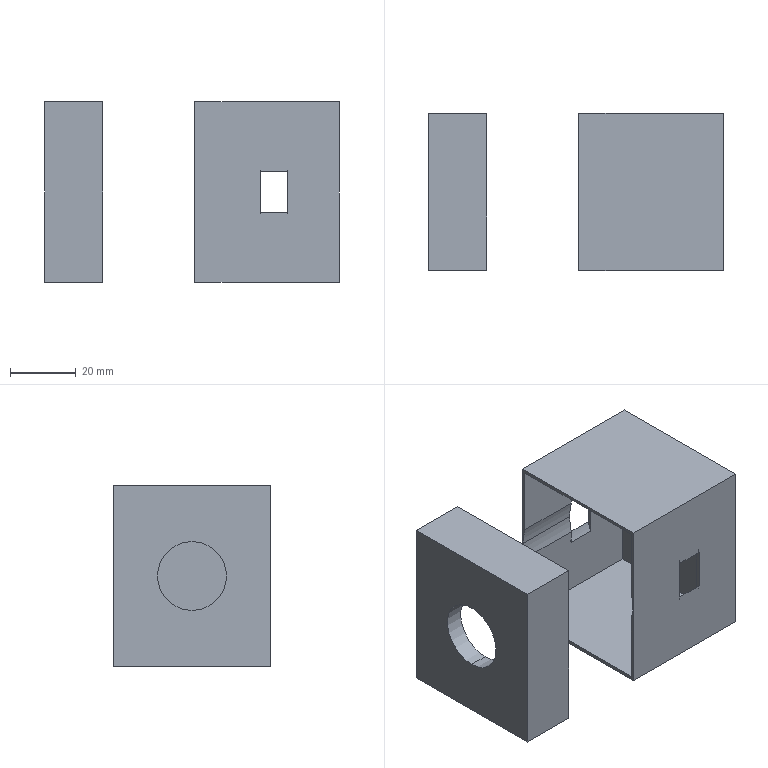Component | SolidWorks | BearingHousing-1 | 2 solids | 35 faces | box 89.77 x 47.79 x 55 mm | volume 28863 mm3 | plane 26 | cylinder 9 | commonest cylinder face diameters 49.4 x4 47.02 x3 21 x2
STEP:
#1=COLOUR_RGB('',0.7922,0.8196,0.9333);
#2=FILL_AREA_STYLE_COLOUR('',#1);
#3=FILL_AREA_STYLE('',(#2));
#4=SURFACE_STYLE_FILL_AREA(#3);
#5=SURFACE_SIDE_STYLE('',(#4));
#6=SURFACE_STYLE_USAGE(.BOTH.,#5);
#7=PRESENTATION_STYLE_ASSIGNMENT((#6));
#8=CARTESIAN_POINT('',(7.824,3.296,-0.0000003));
#9=VERTEX_POINT('',#8);
#10=CARTESIAN_POINT('',(7.824,3.272,-0.2103));
#11=VERTEX_POINT('',#10);
#12=CARTESIAN_POINT('',(7.824,2.371,-0.0000003));
#13=DIRECTION('',(-1.,-0.,-0.));
#14=DIRECTION('',(0.,-1.,-0.));
#15=AXIS2_PLACEMENT_3D('',#12,#13,#14);
#16=CIRCLE('',#15,0.9256);
#17=EDGE_CURVE('',#9,#11,#16,.T.);
#18=ORIENTED_EDGE('',*,*,#17,.F.);
#19=CARTESIAN_POINT('',(7.039,3.296,-0.0000003));
#20=VERTEX_POINT('',#19);
#21=CARTESIAN_POINT('',(7.826,3.296,-0.0000003));
#22=DIRECTION('',(-1.,-0.,-0.));
#23=VECTOR('',#22,39.37);
#24=LINE('',#21,#23);
#25=EDGE_CURVE('',#9,#20,#24,.T.);
#26=ORIENTED_EDGE('',*,*,#25,.T.);
#27=CARTESIAN_POINT('',(7.039,3.272,-0.2103));
#28=VERTEX_POINT('',#27);
#29=CARTESIAN_POINT('',(7.039,2.371,-0.0000003));
#30=DIRECTION('',(-1.,-0.,-0.));
#31=DIRECTION('',(0.,-1.,-0.));
#32=AXIS2_PLACEMENT_3D('',#29,#30,#31);
#33=CIRCLE('',#32,0.9256);
#34=EDGE_CURVE('',#20,#28,#33,.T.);
#35=ORIENTED_EDGE('',*,*,#34,.T.);
#36=CARTESIAN_POINT('',(7.826,3.272,-0.2103));
#37=DIRECTION('',(1.,0.,0.));
#38=VECTOR('',#37,39.37);
#39=LINE('',#36,#38);
#40=EDGE_CURVE('',#28,#11,#39,.T.);
#41=ORIENTED_EDGE('',*,*,#40,.T.);
#42=EDGE_LOOP('',(#18,#26,#35,#41));
#43=FACE_OUTER_BOUND('',#42,.T.);
#44=CARTESIAN_POINT('',(7.826,2.371,-0.0000003));
#45=DIRECTION('',(-1.,-0.,-0.));
#46=DIRECTION('',(0.,1.,0.));
#47=AXIS2_PLACEMENT_3D('',#44,#45,#46);
#48=CYLINDRICAL_SURFACE('',#47,0.9256);
#49=ADVANCED_FACE('',(#43),#48,.F.);
#50=CARTESIAN_POINT('',(7.039,1.469,0.2103));
#51=VERTEX_POINT('',#50);
#52=CARTESIAN_POINT('',(7.824,1.469,0.2103));
#53=VERTEX_POINT('',#52);
#54=CARTESIAN_POINT('',(7.826,1.469,0.2103));
#55=DIRECTION('',(1.,0.,0.));
#56=VECTOR('',#55,39.37);
#57=LINE('',#54,#56);
#58=EDGE_CURVE('',#51,#53,#57,.T.);
#59=ORIENTED_EDGE('',*,*,#58,.F.);
#60=CARTESIAN_POINT('',(7.039,1.469,1.043));
#61=VERTEX_POINT('',#60);
#62=CARTESIAN_POINT('',(7.039,1.469,0.8331));
#63=DIRECTION('',(0.,0.,-1.));
#64=VECTOR('',#63,39.37);
#65=LINE('',#62,#64);
#66=EDGE_CURVE('',#61,#51,#65,.T.);
#67=ORIENTED_EDGE('',*,*,#66,.F.);
#68=CARTESIAN_POINT('',(8.692,1.469,1.043));
#69=VERTEX_POINT('',#68);
#70=CARTESIAN_POINT('',(5.464,1.469,1.043));
#71=DIRECTION('',(1.,0.,0.));
#72=VECTOR('',#71,39.37);
#73=LINE('',#70,#72);
#74=EDGE_CURVE('',#61,#69,#73,.T.);
#75=ORIENTED_EDGE('',*,*,#74,.T.);
#76=CARTESIAN_POINT('',(8.692,1.469,-1.043));
#77=VERTEX_POINT('',#76);
#78=CARTESIAN_POINT('',(8.692,1.469,1.043));
#79=DIRECTION('',(0.,0.,-1.));
#80=VECTOR('',#79,39.37);
#81=LINE('',#78,#80);
#82=EDGE_CURVE('',#69,#77,#81,.T.);
#83=ORIENTED_EDGE('',*,*,#82,.T.);
#84=CARTESIAN_POINT('',(7.039,1.469,-1.043));
#85=VERTEX_POINT('',#84);
#86=CARTESIAN_POINT('',(5.464,1.469,-1.043));
#87=DIRECTION('',(1.,0.,0.));
#88=VECTOR('',#87,39.37);
#89=LINE('',#86,#88);
#90=EDGE_CURVE('',#85,#77,#89,.T.);
#91=ORIENTED_EDGE('',*,*,#90,.F.);
#92=CARTESIAN_POINT('',(7.039,1.469,-0.2103));
#93=VERTEX_POINT('',#92);
#94=CARTESIAN_POINT('',(7.039,1.469,0.8331));
#95=DIRECTION('',(0.,0.,-1.));
#96=VECTOR('',#95,39.37);
#97=LINE('',#94,#96);
#98=EDGE_CURVE('',#93,#85,#97,.T.);
#99=ORIENTED_EDGE('',*,*,#98,.F.);
#100=CARTESIAN_POINT('',(7.824,1.469,-0.2103));
#101=VERTEX_POINT('',#100);
#102=CARTESIAN_POINT('',(7.826,1.469,-0.2103));
#103=DIRECTION('',(-1.,-0.,-0.));
#104=VECTOR('',#103,39.37);
#105=LINE('',#102,#104);
#106=EDGE_CURVE('',#101,#93,#105,.T.);
#107=ORIENTED_EDGE('',*,*,#106,.F.);
#108=CARTESIAN_POINT('',(7.824,1.469,-0.3649));
#109=VERTEX_POINT('',#108);
#110=CARTESIAN_POINT('',(7.824,1.469,1.043));
#111=DIRECTION('',(-0.,-0.,1.));
#112=VECTOR('',#111,39.37);
#113=LINE('',#110,#112);
#114=EDGE_CURVE('',#109,#101,#113,.T.);
#115=ORIENTED_EDGE('',*,*,#114,.F.);
#116=CARTESIAN_POINT('',(8.151,1.469,-0.3649));
#117=VERTEX_POINT('',#116);
#118=CARTESIAN_POINT('',(8.151,1.469,-0.3649));
#119=DIRECTION('',(-1.,-0.,-0.));
#120=VECTOR('',#119,39.37);
#121=LINE('',#118,#120);
#122=EDGE_CURVE('',#117,#109,#121,.T.);
#123=ORIENTED_EDGE('',*,*,#122,.F.);
#124=CARTESIAN_POINT('',(8.151,1.469,0.3649));
#125=VERTEX_POINT('',#124);
#126=CARTESIAN_POINT('',(8.151,1.469,1.043));
#127=DIRECTION('',(-0.,-0.,1.));
#128=VECTOR('',#127,39.37);
#129=LINE('',#126,#128);
#130=EDGE_CURVE('',#117,#125,#129,.T.);
#131=ORIENTED_EDGE('',*,*,#130,.T.);
#132=CARTESIAN_POINT('',(7.824,1.469,0.3649));
#133=VERTEX_POINT('',#132);
#134=CARTESIAN_POINT('',(8.151,1.469,0.3649));
#135=DIRECTION('',(1.,0.,0.));
#136=VECTOR('',#135,39.37);
#137=LINE('',#134,#136);
#138=EDGE_CURVE('',#133,#125,#137,.T.);
#139=ORIENTED_EDGE('',*,*,#138,.F.);
#140=CARTESIAN_POINT('',(7.824,1.469,1.043));
#141=DIRECTION('',(-0.,-0.,1.));
#142=VECTOR('',#141,39.37);
#143=LINE('',#140,#142);
#144=EDGE_CURVE('',#53,#133,#143,.T.);
#145=ORIENTED_EDGE('',*,*,#144,.F.);
#146=EDGE_LOOP('',(#59,#67,#75,#83,#91,#99,#107,#115,#123,#131,#139,#145));
#147=FACE_OUTER_BOUND('',#146,.T.);
#148=CARTESIAN_POINT('',(5.464,1.469,1.043));
#149=DIRECTION('',(0.,-1.,-0.));
#150=DIRECTION('',(0.,0.,-1.));
#151=AXIS2_PLACEMENT_3D('',#148,#149,#150);
#152=PLANE('',#151);
#153=ADVANCED_FACE('',(#147),#152,.F.);
#154=ORIENTED_EDGE('',*,*,#40,.F.);
#155=CARTESIAN_POINT('',(7.039,3.272,-1.043));
#156=VERTEX_POINT('',#155);
#157=CARTESIAN_POINT('',(7.039,3.272,0.8331));
#158=DIRECTION('',(-0.,-0.,1.));
#159=VECTOR('',#158,39.37);
#160=LINE('',#157,#159);
#161=EDGE_CURVE('',#156,#28,#160,.T.);
#162=ORIENTED_EDGE('',*,*,#161,.F.);
#163=CARTESIAN_POINT('',(8.692,3.272,-1.043));
#164=VERTEX_POINT('',#163);
#165=CARTESIAN_POINT('',(5.464,3.272,-1.043));
#166=DIRECTION('',(1.,0.,0.));
#167=VECTOR('',#166,39.37);
#168=LINE('',#165,#167);
#169=EDGE_CURVE('',#156,#164,#168,.T.);
#170=ORIENTED_EDGE('',*,*,#169,.T.);
#171=CARTESIAN_POINT('',(8.692,3.272,1.043));
#172=VERTEX_POINT('',#171);
#173=CARTESIAN_POINT('',(8.692,3.272,-1.043));
#174=DIRECTION('',(-0.,-0.,1.));
#175=VECTOR('',#174,39.37);
#176=LINE('',#173,#175);
#177=EDGE_CURVE('',#164,#172,#176,.T.);
#178=ORIENTED_EDGE('',*,*,#177,.T.);
#179=CARTESIAN_POINT('',(7.039,3.272,1.043));
#180=VERTEX_POINT('',#179);
#181=CARTESIAN_POINT('',(5.464,3.272,1.043));
#182=DIRECTION('',(1.,0.,0.));
#183=VECTOR('',#182,39.37);
#184=LINE('',#181,#183);
#185=EDGE_CURVE('',#180,#172,#184,.T.);
#186=ORIENTED_EDGE('',*,*,#185,.F.);
#187=CARTESIAN_POINT('',(7.039,3.272,0.2103));
#188=VERTEX_POINT('',#187);
#189=CARTESIAN_POINT('',(7.039,3.272,0.8331));
#190=DIRECTION('',(-0.,-0.,1.));
#191=VECTOR('',#190,39.37);
#192=LINE('',#189,#191);
#193=EDGE_CURVE('',#188,#180,#192,.T.);
#194=ORIENTED_EDGE('',*,*,#193,.F.);
#195=CARTESIAN_POINT('',(7.824,3.272,0.2103));
#196=VERTEX_POINT('',#195);
#197=CARTESIAN_POINT('',(7.826,3.272,0.2103));
#198=DIRECTION('',(-1.,-0.,-0.));
#199=VECTOR('',#198,39.37);
#200=LINE('',#197,#199);
#201=EDGE_CURVE('',#196,#188,#200,.T.);
#202=ORIENTED_EDGE('',*,*,#201,.F.);
#203=CARTESIAN_POINT('',(7.824,3.272,0.3649));
#204=VERTEX_POINT('',#203);
#205=CARTESIAN_POINT('',(7.824,3.272,-1.043));
#206=DIRECTION('',(0.,0.,-1.));
#207=VECTOR('',#206,39.37);
#208=LINE('',#205,#207);
#209=EDGE_CURVE('',#204,#196,#208,.T.);
#210=ORIENTED_EDGE('',*,*,#209,.F.);
#211=CARTESIAN_POINT('',(8.151,3.272,0.3649));
#212=VERTEX_POINT('',#211);
#213=CARTESIAN_POINT('',(8.151,3.272,0.3649));
#214=DIRECTION('',(-1.,-0.,-0.));
#215=VECTOR('',#214,39.37);
#216=LINE('',#213,#215);
#217=EDGE_CURVE('',#212,#204,#216,.T.);
#218=ORIENTED_EDGE('',*,*,#217,.F.);
#219=CARTESIAN_POINT('',(8.151,3.272,-0.3649));
#220=VERTEX_POINT('',#219);
#221=CARTESIAN_POINT('',(8.151,3.272,-1.043));
#222=DIRECTION('',(0.,0.,-1.));
#223=VECTOR('',#222,39.37);
#224=LINE('',#221,#223);
#225=EDGE_CURVE('',#212,#220,#224,.T.);
#226=ORIENTED_EDGE('',*,*,#225,.T.);
#227=CARTESIAN_POINT('',(7.824,3.272,-0.3649));
#228=VERTEX_POINT('',#227);
#229=CARTESIAN_POINT('',(8.151,3.272,-0.3649));
#230=DIRECTION('',(1.,0.,0.));
#231=VECTOR('',#230,39.37);
#232=LINE('',#229,#231);
#233=EDGE_CURVE('',#228,#220,#232,.T.);
#234=ORIENTED_EDGE('',*,*,#233,.F.);
#235=CARTESIAN_POINT('',(7.824,3.272,-1.043));
#236=DIRECTION('',(0.,0.,-1.));
#237=VECTOR('',#236,39.37);
#238=LINE('',#235,#237);
#239=EDGE_CURVE('',#11,#228,#238,.T.);
#240=ORIENTED_EDGE('',*,*,#239,.F.);
#241=EDGE_LOOP('',(#154,#162,#170,#178,#186,#194,#202,#210,#218,#226,#234,#240));
#242=FACE_OUTER_BOUND('',#241,.T.);
#243=CARTESIAN_POINT('',(5.464,3.272,-1.043));
#244=DIRECTION('',(-0.,1.,0.));
#245=DIRECTION('',(-0.,-0.,1.));
#246=AXIS2_PLACEMENT_3D('',#243,#244,#245);
#247=PLANE('',#246);
#248=ADVANCED_FACE('',(#242),#247,.F.);
#249=CARTESIAN_POINT('',(7.039,2.371,-0.0000003));
#250=DIRECTION('',(-1.,-0.,-0.));
#251=DIRECTION('',(0.,-1.,-0.));
#252=AXIS2_PLACEMENT_3D('',#249,#250,#251);
#253=CIRCLE('',#252,0.9256);
#254=EDGE_CURVE('',#188,#20,#253,.T.);
#255=ORIENTED_EDGE('',*,*,#254,.F.);
#256=ORIENTED_EDGE('',*,*,#193,.T.);
#257=CARTESIAN_POINT('',(7.039,3.37,1.043));
#258=DIRECTION('',(0.,-1.,-0.));
#259=VECTOR('',#258,39.37);
#260=LINE('',#257,#259);
#261=EDGE_CURVE('',#180,#61,#260,.T.);
#262=ORIENTED_EDGE('',*,*,#261,.T.);
#263=ORIENTED_EDGE('',*,*,#66,.T.);
#264=CARTESIAN_POINT('',(7.039,2.371,-0.0000003));
#265=DIRECTION('',(-1.,-0.,-0.));
#266=DIRECTION('',(0.,-1.,-0.));
#267=AXIS2_PLACEMENT_3D('',#264,#265,#266);
#268=CIRCLE('',#267,0.9256);
#269=EDGE_CURVE('',#93,#51,#268,.T.);
#270=ORIENTED_EDGE('',*,*,#269,.F.);
#271=ORIENTED_EDGE('',*,*,#98,.T.);
#272=CARTESIAN_POINT('',(7.039,3.37,-1.043));
#273=DIRECTION('',(-0.,1.,0.));
#274=VECTOR('',#273,39.37);
#275=LINE('',#272,#274);
#276=EDGE_CURVE('',#85,#156,#275,.T.);
#277=ORIENTED_EDGE('',*,*,#276,.T.);
#278=ORIENTED_EDGE('',*,*,#161,.T.);
#279=ORIENTED_EDGE('',*,*,#34,.F.);
#280=EDGE_LOOP('',(#255,#256,#262,#263,#270,#271,#277,#278,#279));
#281=FACE_BOUND('',#280,.T.);
#282=CARTESIAN_POINT('',(7.039,1.43,1.083));
#283=VERTEX_POINT('',#282);
#284=CARTESIAN_POINT('',(7.039,1.43,-1.083));
#285=VERTEX_POINT('',#284);
#286=CARTESIAN_POINT('',(7.039,1.43,1.083));
#287=DIRECTION('',(0.,0.,-1.));
#288=VECTOR('',#287,39.37);
#289=LINE('',#286,#288);
#290=EDGE_CURVE('',#283,#285,#289,.T.);
#291=ORIENTED_EDGE('',*,*,#290,.F.);
#292=CARTESIAN_POINT('',(7.039,3.312,1.083));
#293=VERTEX_POINT('',#292);
#294=CARTESIAN_POINT('',(7.039,3.312,1.083));
#295=DIRECTION('',(0.,-1.,-0.));
#296=VECTOR('',#295,39.37);
#297=LINE('',#294,#296);
#298=EDGE_CURVE('',#293,#283,#297,.T.);
#299=ORIENTED_EDGE('',*,*,#298,.F.);
#300=CARTESIAN_POINT('',(7.039,3.312,-1.083));
#301=VERTEX_POINT('',#300);
#302=CARTESIAN_POINT('',(7.039,3.312,-1.083));
#303=DIRECTION('',(-0.,-0.,1.));
#304=VECTOR('',#303,39.37);
#305=LINE('',#302,#304);
#306=EDGE_CURVE('',#301,#293,#305,.T.);
#307=ORIENTED_EDGE('',*,*,#306,.F.);
#308=CARTESIAN_POINT('',(7.039,1.43,-1.083));
#309=DIRECTION('',(-0.,1.,0.));
#310=VECTOR('',#309,39.37);
#311=LINE('',#308,#310);
#312=EDGE_CURVE('',#285,#301,#311,.T.);
#313=ORIENTED_EDGE('',*,*,#312,.F.);
#314=EDGE_LOOP('',(#291,#299,#307,#313));
#315=FACE_OUTER_BOUND('',#314,.T.);
#316=CARTESIAN_POINT('',(7.039,3.37,0.8331));
#317=DIRECTION('',(1.,0.,0.));
#318=DIRECTION('',(0.,-1.,-0.));
#319=AXIS2_PLACEMENT_3D('',#316,#317,#318);
#320=PLANE('',#319);
#321=ADVANCED_FACE('',(#281,#315),#320,.F.);
#322=CARTESIAN_POINT('',(8.771,1.43,-1.083));
#323=VERTEX_POINT('',#322);
#324=CARTESIAN_POINT('',(-2.164,1.43,-1.083));
#325=DIRECTION('',(1.,-0.,0.));
#326=VECTOR('',#325,39.37);
#327=LINE('',#324,#326);
#328=EDGE_CURVE('',#285,#323,#327,.T.);
#329=ORIENTED_EDGE('',*,*,#328,.F.);
#330=ORIENTED_EDGE('',*,*,#312,.T.);
#331=CARTESIAN_POINT('',(8.771,3.312,-1.083));
#332=VERTEX_POINT('',#331);
#333=CARTESIAN_POINT('',(-2.164,3.312,-1.083));
#334=DIRECTION('',(-1.,-0.,-0.));
#335=VECTOR('',#334,39.37);
#336=LINE('',#333,#335);
#337=EDGE_CURVE('',#332,#301,#336,.T.);
#338=ORIENTED_EDGE('',*,*,#337,.F.);
#339=CARTESIAN_POINT('',(8.771,1.43,-1.083));
#340=DIRECTION('',(-0.,1.,0.));
#341=VECTOR('',#340,39.37);
#342=LINE('',#339,#341);
#343=EDGE_CURVE('',#323,#332,#342,.T.);
#344=ORIENTED_EDGE('',*,*,#343,.F.);
#345=EDGE_LOOP('',(#329,#330,#338,#344));
#346=FACE_OUTER_BOUND('',#345,.T.);
#347=CARTESIAN_POINT('',(-2.164,3.37,-1.083));
#348=DIRECTION('',(-0.,-0.,1.));
#349=DIRECTION('',(0.,-1.,-0.));
#350=AXIS2_PLACEMENT_3D('',#347,#348,#349);
#351=PLANE('',#350);
#352=ADVANCED_FACE('',(#346),#351,.F.);
#353=ORIENTED_EDGE('',*,*,#298,.T.);
#354=CARTESIAN_POINT('',(8.771,1.43,1.083));
#355=VERTEX_POINT('',#354);
#356=CARTESIAN_POINT('',(-2.164,1.43,1.083));
#357=DIRECTION('',(1.,-0.,0.));
#358=VECTOR('',#357,39.37);
#359=LINE('',#356,#358);
#360=EDGE_CURVE('',#283,#355,#359,.T.);
#361=ORIENTED_EDGE('',*,*,#360,.T.);
#362=CARTESIAN_POINT('',(8.771,3.312,1.083));
#363=VERTEX_POINT('',#362);
#364=CARTESIAN_POINT('',(8.771,3.312,1.083));
#365=DIRECTION('',(0.,-1.,-0.));
#366=VECTOR('',#365,39.37);
#367=LINE('',#364,#366);
#368=EDGE_CURVE('',#363,#355,#367,.T.);
#369=ORIENTED_EDGE('',*,*,#368,.F.);
#370=CARTESIAN_POINT('',(-2.164,3.312,1.083));
#371=DIRECTION('',(-1.,-0.,-0.));
#372=VECTOR('',#371,39.37);
#373=LINE('',#370,#372);
#374=EDGE_CURVE('',#363,#293,#373,.T.);
#375=ORIENTED_EDGE('',*,*,#374,.T.);
#376=EDGE_LOOP('',(#353,#361,#369,#375));
#377=FACE_OUTER_BOUND('',#376,.T.);
#378=CARTESIAN_POINT('',(-2.164,3.37,1.083));
#379=DIRECTION('',(-0.,-0.,1.));
#380=DIRECTION('',(0.,-1.,-0.));
#381=AXIS2_PLACEMENT_3D('',#378,#379,#380);
#382=PLANE('',#381);
#383=ADVANCED_FACE('',(#377),#382,.T.);
#384=CARTESIAN_POINT('',(8.151,1.43,0.2462));
#385=VERTEX_POINT('',#384);
#386=CARTESIAN_POINT('',(7.824,1.43,0.2462));
#387=VERTEX_POINT('',#386);
#388=CARTESIAN_POINT('',(8.151,1.43,0.2462));
#389=DIRECTION('',(-1.,-0.,-0.));
#390=VECTOR('',#389,39.37);
#391=LINE('',#388,#390);
#392=EDGE_CURVE('',#385,#387,#391,.T.);
#393=ORIENTED_EDGE('',*,*,#392,.F.);
#394=CARTESIAN_POINT('',(8.151,1.43,-0.2462));
#395=VERTEX_POINT('',#394);
#396=CARTESIAN_POINT('',(8.151,1.43,1.083));
#397=DIRECTION('',(0.,0.,-1.));
#398=VECTOR('',#397,39.37);
#399=LINE('',#396,#398);
#400=EDGE_CURVE('',#385,#395,#399,.T.);
#401=ORIENTED_EDGE('',*,*,#400,.T.);
#402=CARTESIAN_POINT('',(7.824,1.43,-0.2462));
#403=VERTEX_POINT('',#402);
#404=CARTESIAN_POINT('',(8.151,1.43,-0.2462));
#405=DIRECTION('',(1.,0.,0.));
#406=VECTOR('',#405,39.37);
#407=LINE('',#404,#406);
#408=EDGE_CURVE('',#403,#395,#407,.T.);
#409=ORIENTED_EDGE('',*,*,#408,.F.);
#410=CARTESIAN_POINT('',(7.824,1.43,1.083));
#411=DIRECTION('',(0.,0.,-1.));
#412=VECTOR('',#411,39.37);
#413=LINE('',#410,#412);
#414=EDGE_CURVE('',#387,#403,#413,.T.);
#415=ORIENTED_EDGE('',*,*,#414,.F.);
#416=EDGE_LOOP('',(#393,#401,#409,#415));
#417=FACE_BOUND('',#416,.T.);
#418=ORIENTED_EDGE('',*,*,#360,.F.);
#419=ORIENTED_EDGE('',*,*,#290,.T.);
#420=ORIENTED_EDGE('',*,*,#328,.T.);
#421=CARTESIAN_POINT('',(8.771,1.43,1.083));
#422=DIRECTION('',(0.,0.,-1.));
#423=VECTOR('',#422,39.37);
#424=LINE('',#421,#423);
#425=EDGE_CURVE('',#355,#323,#424,.T.);
#426=ORIENTED_EDGE('',*,*,#425,.F.);
#427=EDGE_LOOP('',(#418,#419,#420,#426));
#428=FACE_OUTER_BOUND('',#427,.T.);
#429=CARTESIAN_POINT('',(-2.164,1.43,1.083));
#430=DIRECTION('',(0.,1.,0.));
#431=DIRECTION('',(-0.,-0.,1.));
#432=AXIS2_PLACEMENT_3D('',#429,#430,#431);
#433=PLANE('',#432);
#434=ADVANCED_FACE('',(#417,#428),#433,.F.);
#435=CARTESIAN_POINT('',(8.151,3.312,-0.2462));
#436=VERTEX_POINT('',#435);
#437=CARTESIAN_POINT('',(7.824,3.312,-0.2462));
#438=VERTEX_POINT('',#437);
#439=CARTESIAN_POINT('',(8.151,3.312,-0.2462));
#440=DIRECTION('',(-1.,-0.,-0.));
#441=VECTOR('',#440,39.37);
#442=LINE('',#439,#441);
#443=EDGE_CURVE('',#436,#438,#442,.T.);
#444=ORIENTED_EDGE('',*,*,#443,.F.);
#445=CARTESIAN_POINT('',(8.151,3.312,0.2462));
#446=VERTEX_POINT('',#445);
#447=CARTESIAN_POINT('',(8.151,3.312,1.083));
#448=DIRECTION('',(-0.,-0.,1.));
#449=VECTOR('',#448,39.37);
#450=LINE('',#447,#449);
#451=EDGE_CURVE('',#436,#446,#450,.T.);
#452=ORIENTED_EDGE('',*,*,#451,.T.);
#453=CARTESIAN_POINT('',(7.824,3.312,0.2462));
#454=VERTEX_POINT('',#453);
#455=CARTESIAN_POINT('',(8.151,3.312,0.2462));
#456=DIRECTION('',(1.,0.,0.));
#457=VECTOR('',#456,39.37);
#458=LINE('',#455,#457);
#459=EDGE_CURVE('',#454,#446,#458,.T.);
#460=ORIENTED_EDGE('',*,*,#459,.F.);
#461=CARTESIAN_POINT('',(7.824,3.312,1.083));
#462=DIRECTION('',(-0.,-0.,1.));
#463=VECTOR('',#462,39.37);
#464=LINE('',#461,#463);
#465=EDGE_CURVE('',#438,#454,#464,.T.);
#466=ORIENTED_EDGE('',*,*,#465,.F.);
#467=EDGE_LOOP('',(#444,#452,#460,#466));
#468=FACE_BOUND('',#467,.T.);
#469=ORIENTED_EDGE('',*,*,#337,.T.);
#470=ORIENTED_EDGE('',*,*,#306,.T.);
#471=ORIENTED_EDGE('',*,*,#374,.F.);
#472=CARTESIAN_POINT('',(8.771,3.312,-1.083));
#473=DIRECTION('',(-0.,-0.,1.));
#474=VECTOR('',#473,39.37);
#475=LINE('',#472,#474);
#476=EDGE_CURVE('',#332,#363,#475,.T.);
#477=ORIENTED_EDGE('',*,*,#476,.F.);
#478=EDGE_LOOP('',(#469,#470,#471,#477));
#479=FACE_OUTER_BOUND('',#478,.T.);
#480=CARTESIAN_POINT('',(-2.164,3.312,1.083));
#481=DIRECTION('',(0.,-1.,-0.));
#482=DIRECTION('',(0.,0.,-1.));
#483=AXIS2_PLACEMENT_3D('',#480,#481,#482);
#484=PLANE('',#483);
#485=ADVANCED_FACE('',(#468,#479),#484,.F.);
#486=CARTESIAN_POINT('',(8.692,3.272,1.043));
#487=DIRECTION('',(0.,-1.,-0.));
#488=VECTOR('',#487,39.37);
#489=LINE('',#486,#488);
#490=EDGE_CURVE('',#172,#69,#489,.T.);
#491=ORIENTED_EDGE('',*,*,#490,.T.);
#492=ORIENTED_EDGE('',*,*,#74,.F.);
#493=ORIENTED_EDGE('',*,*,#261,.F.);
#494=ORIENTED_EDGE('',*,*,#185,.T.);
#495=EDGE_LOOP('',(#491,#492,#493,#494));
#496=FACE_OUTER_BOUND('',#495,.T.);
#497=CARTESIAN_POINT('',(5.464,3.272,1.043));
#498=DIRECTION('',(-0.,-0.,1.));
#499=DIRECTION('',(0.,-1.,-0.));
#500=AXIS2_PLACEMENT_3D('',#497,#498,#499);
#501=PLANE('',#500);
#502=ADVANCED_FACE('',(#496),#501,.F.);
#503=CARTESIAN_POINT('',(8.692,1.469,-1.043));
#504=DIRECTION('',(-0.,1.,0.));
#505=VECTOR('',#504,39.37);
#506=LINE('',#503,#505);
#507=EDGE_CURVE('',#77,#164,#506,.T.);
#508=ORIENTED_EDGE('',*,*,#507,.T.);
#509=ORIENTED_EDGE('',*,*,#169,.F.);
#510=ORIENTED_EDGE('',*,*,#276,.F.);
#511=ORIENTED_EDGE('',*,*,#90,.T.);
#512=EDGE_LOOP('',(#508,#509,#510,#511));
#513=FACE_OUTER_BOUND('',#512,.T.);
#514=CARTESIAN_POINT('',(5.464,1.469,-1.043));
#515=DIRECTION('',(0.,0.,-1.));
#516=DIRECTION('',(-0.,1.,0.));
#517=AXIS2_PLACEMENT_3D('',#514,#515,#516);
#518=PLANE('',#517);
#519=ADVANCED_FACE('',(#513),#518,.F.);
#520=ORIENTED_EDGE('',*,*,#425,.T.);
#521=ORIENTED_EDGE('',*,*,#343,.T.);
#522=ORIENTED_EDGE('',*,*,#476,.T.);
#523=ORIENTED_EDGE('',*,*,#368,.T.);
#524=EDGE_LOOP('',(#520,#521,#522,#523));
#525=FACE_OUTER_BOUND('',#524,.T.);
#526=CARTESIAN_POINT('',(8.771,3.37,0.8331));
#527=DIRECTION('',(1.,0.,0.));
#528=DIRECTION('',(0.,-1.,-0.));
#529=AXIS2_PLACEMENT_3D('',#526,#527,#528);
#530=PLANE('',#529);
#531=ADVANCED_FACE('',(#525),#530,.T.);
#532=ORIENTED_EDGE('',*,*,#490,.F.);
#533=ORIENTED_EDGE('',*,*,#177,.F.);
#534=ORIENTED_EDGE('',*,*,#507,.F.);
#535=ORIENTED_EDGE('',*,*,#82,.F.);
#536=EDGE_LOOP('',(#532,#533,#534,#535));
#537=FACE_OUTER_BOUND('',#536,.T.);
#538=CARTESIAN_POINT('',(8.692,3.37,0.8331));
#539=DIRECTION('',(1.,0.,0.));
#540=DIRECTION('',(0.,-1.,-0.));
#541=AXIS2_PLACEMENT_3D('',#538,#539,#540);
#542=PLANE('',#541);
#543=ADVANCED_FACE('',(#537),#542,.F.);
#544=CARTESIAN_POINT('',(8.151,2.371,-0.0000003));
#545=DIRECTION('',(1.,0.,0.));
#546=DIRECTION('',(0.,-1.,-0.));
#547=AXIS2_PLACEMENT_3D('',#544,#545,#546);
#548=CIRCLE('',#547,0.9724);
#549=EDGE_CURVE('',#220,#436,#548,.T.);
#550=ORIENTED_EDGE('',*,*,#549,.F.);
#551=ORIENTED_EDGE('',*,*,#225,.F.);
#552=CARTESIAN_POINT('',(8.151,2.371,-0.0000003));
#553=DIRECTION('',(1.,0.,0.));
#554=DIRECTION('',(0.,-1.,-0.));
#555=AXIS2_PLACEMENT_3D('',#552,#553,#554);
#556=CIRCLE('',#555,0.9724);
#557=EDGE_CURVE('',#446,#212,#556,.T.);
#558=ORIENTED_EDGE('',*,*,#557,.F.);
#559=ORIENTED_EDGE('',*,*,#451,.F.);
#560=EDGE_LOOP('',(#550,#551,#558,#559));
#561=FACE_OUTER_BOUND('',#560,.T.);
#562=CARTESIAN_POINT('',(8.151,2.371,-0.0000003));
#563=DIRECTION('',(1.,0.,0.));
#564=DIRECTION('',(0.,-1.,-0.));
#565=AXIS2_PLACEMENT_3D('',#562,#563,#564);
#566=PLANE('',#565);
#567=ADVANCED_FACE('',(#561),#566,.F.);
#568=ORIENTED_EDGE('',*,*,#25,.F.);
#569=CARTESIAN_POINT('',(7.824,2.371,-0.0000003));
#570=DIRECTION('',(-1.,-0.,-0.));
#571=DIRECTION('',(0.,-1.,-0.));
#572=AXIS2_PLACEMENT_3D('',#569,#570,#571);
#573=CIRCLE('',#572,0.9256);
#574=EDGE_CURVE('',#196,#9,#573,.T.);
#575=ORIENTED_EDGE('',*,*,#574,.F.);
#576=ORIENTED_EDGE('',*,*,#201,.T.);
#577=ORIENTED_EDGE('',*,*,#254,.T.);
#578=EDGE_LOOP('',(#568,#575,#576,#577));
#579=FACE_OUTER_BOUND('',#578,.T.);
#580=CARTESIAN_POINT('',(7.826,2.371,-0.0000003));
#581=DIRECTION('',(-1.,-0.,-0.));
#582=DIRECTION('',(0.,1.,0.));
#583=AXIS2_PLACEMENT_3D('',#580,#581,#582);
#584=CYLINDRICAL_SURFACE('',#583,0.9256);
#585=ADVANCED_FACE('',(#579),#584,.F.);
#586=ORIENTED_EDGE('',*,*,#465,.T.);
#587=CARTESIAN_POINT('',(7.824,2.371,-0.0000003));
#588=DIRECTION('',(1.,0.,0.));
#589=DIRECTION('',(0.,-1.,-0.));
#590=AXIS2_PLACEMENT_3D('',#587,#588,#589);
#591=CIRCLE('',#590,0.9724);
#592=EDGE_CURVE('',#454,#204,#591,.T.);
#593=ORIENTED_EDGE('',*,*,#592,.T.);
#594=ORIENTED_EDGE('',*,*,#209,.T.);
#595=ORIENTED_EDGE('',*,*,#574,.T.);
#596=ORIENTED_EDGE('',*,*,#17,.T.);
#597=ORIENTED_EDGE('',*,*,#239,.T.);
#598=CARTESIAN_POINT('',(7.824,2.371,-0.0000003));
#599=DIRECTION('',(1.,0.,0.));
#600=DIRECTION('',(0.,-1.,-0.));
#601=AXIS2_PLACEMENT_3D('',#598,#599,#600);
#602=CIRCLE('',#601,0.9724);
#603=EDGE_CURVE('',#228,#438,#602,.T.);
#604=ORIENTED_EDGE('',*,*,#603,.T.);
#605=EDGE_LOOP('',(#586,#593,#594,#595,#596,#597,#604));
#606=FACE_OUTER_BOUND('',#605,.T.);
#607=CARTESIAN_POINT('',(7.824,2.371,-0.0000003));
#608=DIRECTION('',(1.,0.,0.));
#609=DIRECTION('',(0.,-1.,-0.));
#610=AXIS2_PLACEMENT_3D('',#607,#608,#609);
#611=PLANE('',#610);
#612=ADVANCED_FACE('',(#606),#611,.T.);
#613=ORIENTED_EDGE('',*,*,#459,.T.);
#614=ORIENTED_EDGE('',*,*,#557,.T.);
#615=ORIENTED_EDGE('',*,*,#217,.T.);
#616=ORIENTED_EDGE('',*,*,#592,.F.);
#617=EDGE_LOOP('',(#613,#614,#615,#616));
#618=FACE_OUTER_BOUND('',#617,.T.);
#619=CARTESIAN_POINT('',(8.151,2.371,-0.0000003));
#620=DIRECTION('',(-1.,-0.,-0.));
#621=DIRECTION('',(0.,1.,0.));
#622=AXIS2_PLACEMENT_3D('',#619,#620,#621);
#623=CYLINDRICAL_SURFACE('',#622,0.9724);
#624=ADVANCED_FACE('',(#618),#623,.F.);
#625=ORIENTED_EDGE('',*,*,#443,.T.);
#626=ORIENTED_EDGE('',*,*,#603,.F.);
#627=ORIENTED_EDGE('',*,*,#233,.T.);
#628=ORIENTED_EDGE('',*,*,#549,.T.);
#629=EDGE_LOOP('',(#625,#626,#627,#628));
#630=FACE_OUTER_BOUND('',#629,.T.);
#631=CARTESIAN_POINT('',(8.151,2.371,-0.0000003));
#632=DIRECTION('',(-1.,-0.,-0.));
#633=DIRECTION('',(0.,1.,0.));
#634=AXIS2_PLACEMENT_3D('',#631,#632,#633);
#635=CYLINDRICAL_SURFACE('',#634,0.9724);
#636=ADVANCED_FACE('',(#630),#635,.F.);
#637=ORIENTED_EDGE('',*,*,#408,.T.);
#638=CARTESIAN_POINT('',(8.151,2.371,-0.0000003));
#639=DIRECTION('',(1.,0.,0.));
#640=DIRECTION('',(0.,-1.,-0.));
#641=AXIS2_PLACEMENT_3D('',#638,#639,#640);
#642=CIRCLE('',#641,0.9724);
#643=EDGE_CURVE('',#395,#117,#642,.T.);
#644=ORIENTED_EDGE('',*,*,#643,.T.);
#645=ORIENTED_EDGE('',*,*,#122,.T.);
#646=CARTESIAN_POINT('',(7.824,2.371,-0.0000003));
#647=DIRECTION('',(1.,0.,0.));
#648=DIRECTION('',(0.,-1.,-0.));
#649=AXIS2_PLACEMENT_3D('',#646,#647,#648);
#650=CIRCLE('',#649,0.9724);
#651=EDGE_CURVE('',#403,#109,#650,.T.);
#652=ORIENTED_EDGE('',*,*,#651,.F.);
#653=EDGE_LOOP('',(#637,#644,#645,#652));
#654=FACE_OUTER_BOUND('',#653,.T.);
#655=CARTESIAN_POINT('',(8.151,2.371,-0.0000003));
#656=DIRECTION('',(-1.,-0.,-0.));
#657=DIRECTION('',(0.,1.,0.));
#658=AXIS2_PLACEMENT_3D('',#655,#656,#657);
#659=CYLINDRICAL_SURFACE('',#658,0.9724);
#660=ADVANCED_FACE('',(#654),#659,.F.);
#661=ORIENTED_EDGE('',*,*,#392,.T.);
#662=CARTESIAN_POINT('',(7.824,2.371,-0.0000003));
#663=DIRECTION('',(1.,0.,0.));
#664=DIRECTION('',(0.,-1.,-0.));
#665=AXIS2_PLACEMENT_3D('',#662,#663,#664);
#666=CIRCLE('',#665,0.9724);
#667=EDGE_CURVE('',#133,#387,#666,.T.);
#668=ORIENTED_EDGE('',*,*,#667,.F.);
#669=ORIENTED_EDGE('',*,*,#138,.T.);
#670=CARTESIAN_POINT('',(8.151,2.371,-0.0000003));
#671=DIRECTION('',(1.,0.,0.));
#672=DIRECTION('',(0.,-1.,-0.));
#673=AXIS2_PLACEMENT_3D('',#670,#671,#672);
#674=CIRCLE('',#673,0.9724);
#675=EDGE_CURVE('',#125,#385,#674,.T.);
#676=ORIENTED_EDGE('',*,*,#675,.T.);
#677=EDGE_LOOP('',(#661,#668,#669,#676));
#678=FACE_OUTER_BOUND('',#677,.T.);
#679=CARTESIAN_POINT('',(8.151,2.371,-0.0000003));
#680=DIRECTION('',(-1.,-0.,-0.));
#681=DIRECTION('',(0.,1.,0.));
#682=AXIS2_PLACEMENT_3D('',#679,#680,#681);
#683=CYLINDRICAL_SURFACE('',#682,0.9724);
#684=ADVANCED_FACE('',(#678),#683,.F.);
#685=ORIENTED_EDGE('',*,*,#675,.F.);
#686=ORIENTED_EDGE('',*,*,#130,.F.);
#687=ORIENTED_EDGE('',*,*,#643,.F.);
#688=ORIENTED_EDGE('',*,*,#400,.F.);
#689=EDGE_LOOP('',(#685,#686,#687,#688));
#690=FACE_OUTER_BOUND('',#689,.T.);
#691=CARTESIAN_POINT('',(8.151,2.371,-0.0000003));
#692=DIRECTION('',(1.,0.,0.));
#693=DIRECTION('',(0.,-1.,-0.));
#694=AXIS2_PLACEMENT_3D('',#691,#692,#693);
#695=PLANE('',#694);
#696=ADVANCED_FACE('',(#690),#695,.F.);
#697=ORIENTED_EDGE('',*,*,#414,.T.);
#698=ORIENTED_EDGE('',*,*,#651,.T.);
#699=ORIENTED_EDGE('',*,*,#114,.T.);
#700=CARTESIAN_POINT('',(7.824,2.371,-0.0000003));
#701=DIRECTION('',(-1.,-0.,-0.));
#702=DIRECTION('',(0.,-1.,-0.));
#703=AXIS2_PLACEMENT_3D('',#700,#701,#702);
#704=CIRCLE('',#703,0.9256);
#705=EDGE_CURVE('',#101,#53,#704,.T.);
#706=ORIENTED_EDGE('',*,*,#705,.T.);
#707=ORIENTED_EDGE('',*,*,#144,.T.);
#708=ORIENTED_EDGE('',*,*,#667,.T.);
#709=EDGE_LOOP('',(#697,#698,#699,#706,#707,#708));
#710=FACE_OUTER_BOUND('',#709,.T.);
#711=CARTESIAN_POINT('',(7.824,2.371,-0.0000003));
#712=DIRECTION('',(1.,0.,0.));
#713=DIRECTION('',(0.,-1.,-0.));
#714=AXIS2_PLACEMENT_3D('',#711,#712,#713);
#715=PLANE('',#714);
#716=ADVANCED_FACE('',(#710),#715,.T.);
#717=ORIENTED_EDGE('',*,*,#58,.T.);
#718=ORIENTED_EDGE('',*,*,#705,.F.);
#719=ORIENTED_EDGE('',*,*,#106,.T.);
#720=ORIENTED_EDGE('',*,*,#269,.T.);
#721=EDGE_LOOP('',(#717,#718,#719,#720));
#722=FACE_OUTER_BOUND('',#721,.T.);
#723=CARTESIAN_POINT('',(7.826,2.371,-0.0000003));
#724=DIRECTION('',(-1.,-0.,-0.));
#725=DIRECTION('',(0.,1.,0.));
#726=AXIS2_PLACEMENT_3D('',#723,#724,#725);
#727=CYLINDRICAL_SURFACE('',#726,0.9256);
#728=ADVANCED_FACE('',(#722),#727,.F.);
#729=CLOSED_SHELL('',(#49,#153,#248,#321,#352,#383,#434,#485,#502,#519,#531,#543,#567,#585,#612,#624,#636,#660,#684,#696,#716,#728));
#730=MANIFOLD_SOLID_BREP('',#729);
#731=STYLED_ITEM('',(#7),#730);
#732=(LENGTH_UNIT()NAMED_UNIT(*)SI_UNIT($,.METRE.));
#733=LENGTH_MEASURE_WITH_UNIT(LENGTH_MEASURE(0.0254),#732);
#734=DIMENSIONAL_EXPONENTS(1.,0.,0.,0.,0.,0.,0.);
#735=(CONVERSION_BASED_UNIT('',#733)LENGTH_UNIT()NAMED_UNIT(#734));
#736=UNCERTAINTY_MEASURE_WITH_UNIT(LENGTH_MEASURE(0.00001),#735,'','');
#737=(NAMED_UNIT(*)PLANE_ANGLE_UNIT()SI_UNIT($,.RADIAN.));
#738=(NAMED_UNIT(*)SI_UNIT($,.STERADIAN.)SOLID_ANGLE_UNIT());
#739=(GEOMETRIC_REPRESENTATION_CONTEXT(3)GLOBAL_UNCERTAINTY_ASSIGNED_CONTEXT((#736))GLOBAL_UNIT_ASSIGNED_CONTEXT((#735,#737,#738))REPRESENTATION_CONTEXT('',''));
#740=MECHANICAL_DESIGN_GEOMETRIC_PRESENTATION_REPRESENTATION('',(#731),#739);
#741=COLOUR_RGB('',0.7922,0.8196,0.9333);
#742=FILL_AREA_STYLE_COLOUR('',#741);
#743=FILL_AREA_STYLE('',(#742));
#744=SURFACE_STYLE_FILL_AREA(#743);
#745=SURFACE_SIDE_STYLE('',(#744));
#746=SURFACE_STYLE_USAGE(.BOTH.,#745);
#747=PRESENTATION_STYLE_ASSIGNMENT((#746));
#748=CARTESIAN_POINT('',(5.464,2.371,-0.4134));
#749=VERTEX_POINT('',#748);
#750=CARTESIAN_POINT('',(5.464,2.371,0.4134));
#751=VERTEX_POINT('',#750);
#752=CARTESIAN_POINT('',(5.464,2.371,-0.));
#753=DIRECTION('',(-1.,-0.,-0.));
#754=DIRECTION('',(0.,-1.,-0.));
#755=AXIS2_PLACEMENT_3D('',#752,#753,#754);
#756=CIRCLE('',#755,0.4134);
#757=EDGE_CURVE('',#749,#751,#756,.T.);
#758=ORIENTED_EDGE('',*,*,#757,.F.);
#759=CARTESIAN_POINT('',(5.237,2.371,-0.4134));
#760=VERTEX_POINT('',#759);
#761=CARTESIAN_POINT('',(7.639,2.371,-0.4134));
#762=DIRECTION('',(-1.,-0.,-0.));
#763=VECTOR('',#762,39.37);
#764=LINE('',#761,#763);
#765=EDGE_CURVE('',#749,#760,#764,.T.);
#766=ORIENTED_EDGE('',*,*,#765,.T.);
#767=CARTESIAN_POINT('',(5.237,2.371,0.4134));
#768=VERTEX_POINT('',#767);
#769=CARTESIAN_POINT('',(5.237,2.371,-0.));
#770=DIRECTION('',(-1.,-0.,-0.));
#771=DIRECTION('',(0.,-0.,1.));
#772=AXIS2_PLACEMENT_3D('',#769,#770,#771);
#773=CIRCLE('',#772,0.4134);
#774=EDGE_CURVE('',#760,#768,#773,.T.);
#775=ORIENTED_EDGE('',*,*,#774,.T.);
#776=CARTESIAN_POINT('',(7.639,2.371,0.4134));
#777=DIRECTION('',(-1.,-0.,-0.));
#778=VECTOR('',#777,39.37);
#779=LINE('',#776,#778);
#780=EDGE_CURVE('',#751,#768,#779,.T.);
#781=ORIENTED_EDGE('',*,*,#780,.F.);
#782=EDGE_LOOP('',(#758,#766,#775,#781));
#783=FACE_OUTER_BOUND('',#782,.T.);
#784=CARTESIAN_POINT('',(7.639,2.371,-0.));
#785=DIRECTION('',(-1.,-0.,-0.));
#786=DIRECTION('',(0.,-0.,1.));
#787=AXIS2_PLACEMENT_3D('',#784,#785,#786);
#788=CYLINDRICAL_SURFACE('',#787,0.4134);
#789=ADVANCED_FACE('',(#783),#788,.F.);
#790=CARTESIAN_POINT('',(5.237,1.43,1.083));
#791=VERTEX_POINT('',#790);
#792=CARTESIAN_POINT('',(5.936,1.43,1.083));
#793=VERTEX_POINT('',#792);
#794=CARTESIAN_POINT('',(-2.164,1.43,1.083));
#795=DIRECTION('',(1.,-0.,0.));
#796=VECTOR('',#795,39.37);
#797=LINE('',#794,#796);
#798=EDGE_CURVE('',#791,#793,#797,.T.);
#799=ORIENTED_EDGE('',*,*,#798,.T.);
#800=CARTESIAN_POINT('',(5.936,3.312,1.083));
#801=VERTEX_POINT('',#800);
#802=CARTESIAN_POINT('',(5.936,3.312,1.083));
#803=DIRECTION('',(0.,-1.,-0.));
#804=VECTOR('',#803,39.37);
#805=LINE('',#802,#804);
#806=EDGE_CURVE('',#801,#793,#805,.T.);
#807=ORIENTED_EDGE('',*,*,#806,.F.);
#808=CARTESIAN_POINT('',(5.237,3.312,1.083));
#809=VERTEX_POINT('',#808);
#810=CARTESIAN_POINT('',(-2.164,3.312,1.083));
#811=DIRECTION('',(-1.,-0.,-0.));
#812=VECTOR('',#811,39.37);
#813=LINE('',#810,#812);
#814=EDGE_CURVE('',#801,#809,#813,.T.);
#815=ORIENTED_EDGE('',*,*,#814,.T.);
#816=CARTESIAN_POINT('',(5.237,3.37,1.083));
#817=DIRECTION('',(0.,-1.,-0.));
#818=VECTOR('',#817,39.37);
#819=LINE('',#816,#818);
#820=EDGE_CURVE('',#809,#791,#819,.T.);
#821=ORIENTED_EDGE('',*,*,#820,.T.);
#822=EDGE_LOOP('',(#799,#807,#815,#821));
#823=FACE_OUTER_BOUND('',#822,.T.);
#824=CARTESIAN_POINT('',(-2.164,3.37,1.083));
#825=DIRECTION('',(-0.,-0.,1.));
#826=DIRECTION('',(0.,-1.,-0.));
#827=AXIS2_PLACEMENT_3D('',#824,#825,#826);
#828=PLANE('',#827);
#829=ADVANCED_FACE('',(#823),#828,.T.);
#830=CARTESIAN_POINT('',(5.936,3.312,-1.083));
#831=VERTEX_POINT('',#830);
#832=CARTESIAN_POINT('',(5.936,3.312,-1.083));
#833=DIRECTION('',(-0.,-0.,1.));
#834=VECTOR('',#833,39.37);
#835=LINE('',#832,#834);
#836=EDGE_CURVE('',#831,#801,#835,.T.);
#837=ORIENTED_EDGE('',*,*,#836,.F.);
#838=CARTESIAN_POINT('',(5.237,3.312,-1.083));
#839=VERTEX_POINT('',#838);
#840=CARTESIAN_POINT('',(-2.164,3.312,-1.083));
#841=DIRECTION('',(-1.,-0.,-0.));
#842=VECTOR('',#841,39.37);
#843=LINE('',#840,#842);
#844=EDGE_CURVE('',#831,#839,#843,.T.);
#845=ORIENTED_EDGE('',*,*,#844,.T.);
#846=CARTESIAN_POINT('',(5.237,3.312,1.083));
#847=DIRECTION('',(0.,0.,-1.));
#848=VECTOR('',#847,39.37);
#849=LINE('',#846,#848);
#850=EDGE_CURVE('',#809,#839,#849,.T.);
#851=ORIENTED_EDGE('',*,*,#850,.F.);
#852=ORIENTED_EDGE('',*,*,#814,.F.);
#853=EDGE_LOOP('',(#837,#845,#851,#852));
#854=FACE_OUTER_BOUND('',#853,.T.);
#855=CARTESIAN_POINT('',(-2.164,3.312,1.083));
#856=DIRECTION('',(0.,-1.,-0.));
#857=DIRECTION('',(0.,0.,-1.));
#858=AXIS2_PLACEMENT_3D('',#855,#856,#857);
#859=PLANE('',#858);
#860=ADVANCED_FACE('',(#854),#859,.F.);
#861=CARTESIAN_POINT('',(5.936,1.43,-1.083));
#862=VERTEX_POINT('',#861);
#863=CARTESIAN_POINT('',(5.936,1.43,-1.083));
#864=DIRECTION('',(-0.,1.,0.));
#865=VECTOR('',#864,39.37);
#866=LINE('',#863,#865);
#867=EDGE_CURVE('',#862,#831,#866,.T.);
#868=ORIENTED_EDGE('',*,*,#867,.F.);
#869=CARTESIAN_POINT('',(5.237,1.43,-1.083));
#870=VERTEX_POINT('',#869);
#871=CARTESIAN_POINT('',(-2.164,1.43,-1.083));
#872=DIRECTION('',(1.,-0.,0.));
#873=VECTOR('',#872,39.37);
#874=LINE('',#871,#873);
#875=EDGE_CURVE('',#870,#862,#874,.T.);
#876=ORIENTED_EDGE('',*,*,#875,.F.);
#877=CARTESIAN_POINT('',(5.237,3.37,-1.083));
#878=DIRECTION('',(0.,-1.,-0.));
#879=VECTOR('',#878,39.37);
#880=LINE('',#877,#879);
#881=EDGE_CURVE('',#839,#870,#880,.T.);
#882=ORIENTED_EDGE('',*,*,#881,.F.);
#883=ORIENTED_EDGE('',*,*,#844,.F.);
#884=EDGE_LOOP('',(#868,#876,#882,#883));
#885=FACE_OUTER_BOUND('',#884,.T.);
#886=CARTESIAN_POINT('',(-2.164,3.37,-1.083));
#887=DIRECTION('',(-0.,-0.,1.));
#888=DIRECTION('',(0.,-1.,-0.));
#889=AXIS2_PLACEMENT_3D('',#886,#887,#888);
#890=PLANE('',#889);
#891=ADVANCED_FACE('',(#885),#890,.F.);
#892=CARTESIAN_POINT('',(5.237,2.371,-0.));
#893=DIRECTION('',(-1.,-0.,-0.));
#894=DIRECTION('',(0.,-0.,1.));
#895=AXIS2_PLACEMENT_3D('',#892,#893,#894);
#896=CIRCLE('',#895,0.4134);
#897=EDGE_CURVE('',#768,#760,#896,.T.);
#898=ORIENTED_EDGE('',*,*,#897,.F.);
#899=ORIENTED_EDGE('',*,*,#774,.F.);
#900=EDGE_LOOP('',(#898,#899));
#901=FACE_BOUND('',#900,.T.);
#902=ORIENTED_EDGE('',*,*,#881,.T.);
#903=CARTESIAN_POINT('',(5.237,1.43,1.083));
#904=DIRECTION('',(0.,0.,-1.));
#905=VECTOR('',#904,39.37);
#906=LINE('',#903,#905);
#907=EDGE_CURVE('',#791,#870,#906,.T.);
#908=ORIENTED_EDGE('',*,*,#907,.F.);
#909=ORIENTED_EDGE('',*,*,#820,.F.);
#910=ORIENTED_EDGE('',*,*,#850,.T.);
#911=EDGE_LOOP('',(#902,#908,#909,#910));
#912=FACE_OUTER_BOUND('',#911,.T.);
#913=CARTESIAN_POINT('',(5.237,3.37,1.083));
#914=DIRECTION('',(1.,0.,0.));
#915=DIRECTION('',(0.,0.,-1.));
#916=AXIS2_PLACEMENT_3D('',#913,#914,#915);
#917=PLANE('',#916);
#918=ADVANCED_FACE('',(#901,#912),#917,.F.);
#919=ORIENTED_EDGE('',*,*,#765,.F.);
#920=CARTESIAN_POINT('',(5.464,2.371,-0.));
#921=DIRECTION('',(-1.,-0.,-0.));
#922=DIRECTION('',(0.,-1.,-0.));
#923=AXIS2_PLACEMENT_3D('',#920,#921,#922);
#924=CIRCLE('',#923,0.4134);
#925=EDGE_CURVE('',#751,#749,#924,.T.);
#926=ORIENTED_EDGE('',*,*,#925,.F.);
#927=ORIENTED_EDGE('',*,*,#780,.T.);
#928=ORIENTED_EDGE('',*,*,#897,.T.);
#929=EDGE_LOOP('',(#919,#926,#927,#928));
#930=FACE_OUTER_BOUND('',#929,.T.);
#931=CARTESIAN_POINT('',(7.639,2.371,-0.));
#932=DIRECTION('',(-1.,-0.,-0.));
#933=DIRECTION('',(0.,-0.,1.));
#934=AXIS2_PLACEMENT_3D('',#931,#932,#933);
#935=CYLINDRICAL_SURFACE('',#934,0.4134);
#936=ADVANCED_FACE('',(#930),#935,.F.);
#937=CARTESIAN_POINT('',(5.936,1.43,1.083));
#938=DIRECTION('',(0.,0.,-1.));
#939=VECTOR('',#938,39.37);
#940=LINE('',#937,#939);
#941=EDGE_CURVE('',#793,#862,#940,.T.);
#942=ORIENTED_EDGE('',*,*,#941,.F.);
#943=ORIENTED_EDGE('',*,*,#798,.F.);
#944=ORIENTED_EDGE('',*,*,#907,.T.);
#945=ORIENTED_EDGE('',*,*,#875,.T.);
#946=EDGE_LOOP('',(#942,#943,#944,#945));
#947=FACE_OUTER_BOUND('',#946,.T.);
#948=CARTESIAN_POINT('',(-2.164,1.43,1.083));
#949=DIRECTION('',(0.,1.,0.));
#950=DIRECTION('',(-0.,-0.,1.));
#951=AXIS2_PLACEMENT_3D('',#948,#949,#950);
#952=PLANE('',#951);
#953=ADVANCED_FACE('',(#947),#952,.F.);
#954=CARTESIAN_POINT('',(5.936,1.469,1.043));
#955=VERTEX_POINT('',#954);
#956=CARTESIAN_POINT('',(5.936,1.469,-1.043));
#957=VERTEX_POINT('',#956);
#958=CARTESIAN_POINT('',(5.936,1.469,0.8331));
#959=DIRECTION('',(0.,0.,-1.));
#960=VECTOR('',#959,39.37);
#961=LINE('',#958,#960);
#962=EDGE_CURVE('',#955,#957,#961,.T.);
#963=ORIENTED_EDGE('',*,*,#962,.F.);
#964=CARTESIAN_POINT('',(5.936,3.272,1.043));
#965=VERTEX_POINT('',#964);
#966=CARTESIAN_POINT('',(5.936,3.37,1.043));
#967=DIRECTION('',(0.,-1.,-0.));
#968=VECTOR('',#967,39.37);
#969=LINE('',#966,#968);
#970=EDGE_CURVE('',#965,#955,#969,.T.);
#971=ORIENTED_EDGE('',*,*,#970,.F.);
#972=CARTESIAN_POINT('',(5.936,3.272,-1.043));
#973=VERTEX_POINT('',#972);
#974=CARTESIAN_POINT('',(5.936,3.272,0.8331));
#975=DIRECTION('',(-0.,-0.,1.));
#976=VECTOR('',#975,39.37);
#977=LINE('',#974,#976);
#978=EDGE_CURVE('',#973,#965,#977,.T.);
#979=ORIENTED_EDGE('',*,*,#978,.F.);
#980=CARTESIAN_POINT('',(5.936,3.37,-1.043));
#981=DIRECTION('',(-0.,1.,0.));
#982=VECTOR('',#981,39.37);
#983=LINE('',#980,#982);
#984=EDGE_CURVE('',#957,#973,#983,.T.);
#985=ORIENTED_EDGE('',*,*,#984,.F.);
#986=EDGE_LOOP('',(#963,#971,#979,#985));
#987=FACE_BOUND('',#986,.T.);
#988=ORIENTED_EDGE('',*,*,#941,.T.);
#989=ORIENTED_EDGE('',*,*,#867,.T.);
#990=ORIENTED_EDGE('',*,*,#836,.T.);
#991=ORIENTED_EDGE('',*,*,#806,.T.);
#992=EDGE_LOOP('',(#988,#989,#990,#991));
#993=FACE_OUTER_BOUND('',#992,.T.);
#994=CARTESIAN_POINT('',(5.936,3.37,0.8331));
#995=DIRECTION('',(1.,0.,0.));
#996=DIRECTION('',(0.,-1.,-0.));
#997=AXIS2_PLACEMENT_3D('',#994,#995,#996);
#998=PLANE('',#997);
#999=ADVANCED_FACE('',(#987,#993),#998,.T.);
#1000=CARTESIAN_POINT('',(5.464,1.469,1.043));
#1001=VERTEX_POINT('',#1000);
#1002=CARTESIAN_POINT('',(5.464,1.469,-1.043));
#1003=VERTEX_POINT('',#1002);
#1004=CARTESIAN_POINT('',(5.464,1.469,1.043));
#1005=DIRECTION('',(0.,0.,-1.));
#1006=VECTOR('',#1005,39.37);
#1007=LINE('',#1004,#1006);
#1008=EDGE_CURVE('',#1001,#1003,#1007,.T.);
#1009=ORIENTED_EDGE('',*,*,#1008,.T.);
#1010=CARTESIAN_POINT('',(5.464,3.272,-1.043));
#1011=VERTEX_POINT('',#1010);
#1012=CARTESIAN_POINT('',(5.464,1.469,-1.043));
#1013=DIRECTION('',(-0.,1.,0.));
#1014=VECTOR('',#1013,39.37);
#1015=LINE('',#1012,#1014);
#1016=EDGE_CURVE('',#1003,#1011,#1015,.T.);
#1017=ORIENTED_EDGE('',*,*,#1016,.T.);
#1018=CARTESIAN_POINT('',(5.464,3.272,1.043));
#1019=VERTEX_POINT('',#1018);
#1020=CARTESIAN_POINT('',(5.464,3.272,-1.043));
#1021=DIRECTION('',(-0.,-0.,1.));
#1022=VECTOR('',#1021,39.37);
#1023=LINE('',#1020,#1022);
#1024=EDGE_CURVE('',#1011,#1019,#1023,.T.);
#1025=ORIENTED_EDGE('',*,*,#1024,.T.);
#1026=CARTESIAN_POINT('',(5.464,3.272,1.043));
#1027=DIRECTION('',(0.,-1.,-0.));
#1028=VECTOR('',#1027,39.37);
#1029=LINE('',#1026,#1028);
#1030=EDGE_CURVE('',#1019,#1001,#1029,.T.);
#1031=ORIENTED_EDGE('',*,*,#1030,.T.);
#1032=EDGE_LOOP('',(#1009,#1017,#1025,#1031));
#1033=FACE_OUTER_BOUND('',#1032,.T.);
#1034=ORIENTED_EDGE('',*,*,#925,.T.);
#1035=ORIENTED_EDGE('',*,*,#757,.T.);
#1036=EDGE_LOOP('',(#1034,#1035));
#1037=FACE_BOUND('',#1036,.T.);
#1038=CARTESIAN_POINT('',(5.464,3.37,0.8331));
#1039=DIRECTION('',(1.,0.,0.));
#1040=DIRECTION('',(0.,-1.,-0.));
#1041=AXIS2_PLACEMENT_3D('',#1038,#1039,#1040);
#1042=PLANE('',#1041);
#1043=ADVANCED_FACE('',(#1033,#1037),#1042,.T.);
#1044=ORIENTED_EDGE('',*,*,#984,.T.);
#1045=CARTESIAN_POINT('',(5.464,3.272,-1.043));
#1046=DIRECTION('',(1.,0.,0.));
#1047=VECTOR('',#1046,39.37);
#1048=LINE('',#1045,#1047);
#1049=EDGE_CURVE('',#1011,#973,#1048,.T.);
#1050=ORIENTED_EDGE('',*,*,#1049,.F.);
#1051=ORIENTED_EDGE('',*,*,#1016,.F.);
#1052=CARTESIAN_POINT('',(5.464,1.469,-1.043));
#1053=DIRECTION('',(1.,0.,0.));
#1054=VECTOR('',#1053,39.37);
#1055=LINE('',#1052,#1054);
#1056=EDGE_CURVE('',#1003,#957,#1055,.T.);
#1057=ORIENTED_EDGE('',*,*,#1056,.T.);
#1058=EDGE_LOOP('',(#1044,#1050,#1051,#1057));
#1059=FACE_OUTER_BOUND('',#1058,.T.);
#1060=CARTESIAN_POINT('',(5.464,1.469,-1.043));
#1061=DIRECTION('',(0.,0.,-1.));
#1062=DIRECTION('',(-0.,1.,0.));
#1063=AXIS2_PLACEMENT_3D('',#1060,#1061,#1062);
#1064=PLANE('',#1063);
#1065=ADVANCED_FACE('',(#1059),#1064,.F.);
#1066=ORIENTED_EDGE('',*,*,#978,.T.);
#1067=CARTESIAN_POINT('',(5.464,3.272,1.043));
#1068=DIRECTION('',(1.,0.,0.));
#1069=VECTOR('',#1068,39.37);
#1070=LINE('',#1067,#1069);
#1071=EDGE_CURVE('',#1019,#965,#1070,.T.);
#1072=ORIENTED_EDGE('',*,*,#1071,.F.);
#1073=ORIENTED_EDGE('',*,*,#1024,.F.);
#1074=ORIENTED_EDGE('',*,*,#1049,.T.);
#1075=EDGE_LOOP('',(#1066,#1072,#1073,#1074));
#1076=FACE_OUTER_BOUND('',#1075,.T.);
#1077=CARTESIAN_POINT('',(5.464,3.272,-1.043));
#1078=DIRECTION('',(-0.,1.,0.));
#1079=DIRECTION('',(-0.,-0.,1.));
#1080=AXIS2_PLACEMENT_3D('',#1077,#1078,#1079);
#1081=PLANE('',#1080);
#1082=ADVANCED_FACE('',(#1076),#1081,.F.);
#1083=ORIENTED_EDGE('',*,*,#970,.T.);
#1084=CARTESIAN_POINT('',(5.464,1.469,1.043));
#1085=DIRECTION('',(1.,0.,0.));
#1086=VECTOR('',#1085,39.37);
#1087=LINE('',#1084,#1086);
#1088=EDGE_CURVE('',#1001,#955,#1087,.T.);
#1089=ORIENTED_EDGE('',*,*,#1088,.F.);
#1090=ORIENTED_EDGE('',*,*,#1030,.F.);
#1091=ORIENTED_EDGE('',*,*,#1071,.T.);
#1092=EDGE_LOOP('',(#1083,#1089,#1090,#1091));
#1093=FACE_OUTER_BOUND('',#1092,.T.);
#1094=CARTESIAN_POINT('',(5.464,3.272,1.043));
#1095=DIRECTION('',(-0.,-0.,1.));
#1096=DIRECTION('',(0.,-1.,-0.));
#1097=AXIS2_PLACEMENT_3D('',#1094,#1095,#1096);
#1098=PLANE('',#1097);
#1099=ADVANCED_FACE('',(#1093),#1098,.F.);
#1100=ORIENTED_EDGE('',*,*,#962,.T.);
#1101=ORIENTED_EDGE('',*,*,#1056,.F.);
#1102=ORIENTED_EDGE('',*,*,#1008,.F.);
#1103=ORIENTED_EDGE('',*,*,#1088,.T.);
#1104=EDGE_LOOP('',(#1100,#1101,#1102,#1103));
#1105=FACE_OUTER_BOUND('',#1104,.T.);
#1106=CARTESIAN_POINT('',(5.464,1.469,1.043));
#1107=DIRECTION('',(0.,-1.,-0.));
#1108=DIRECTION('',(0.,0.,-1.));
#1109=AXIS2_PLACEMENT_3D('',#1106,#1107,#1108);
#1110=PLANE('',#1109);
#1111=ADVANCED_FACE('',(#1105),#1110,.F.);
#1112=CLOSED_SHELL('',(#789,#829,#860,#891,#918,#936,#953,#999,#1043,#1065,#1082,#1099,#1111));
#1113=MANIFOLD_SOLID_BREP('',#1112);
#1114=STYLED_ITEM('',(#747),#1113);
#1115=(LENGTH_UNIT()NAMED_UNIT(*)SI_UNIT($,.METRE.));
#1116=LENGTH_MEASURE_WITH_UNIT(LENGTH_MEASURE(0.0254),#1115);
#1117=DIMENSIONAL_EXPONENTS(1.,0.,0.,0.,0.,0.,0.);
#1118=(CONVERSION_BASED_UNIT('',#1116)LENGTH_UNIT()NAMED_UNIT(#1117));
#1119=UNCERTAINTY_MEASURE_WITH_UNIT(LENGTH_MEASURE(0.00001),#1118,'','');
#1120=(NAMED_UNIT(*)PLANE_ANGLE_UNIT()SI_UNIT($,.RADIAN.));
#1121=(NAMED_UNIT(*)SI_UNIT($,.STERADIAN.)SOLID_ANGLE_UNIT());
#1122=(GEOMETRIC_REPRESENTATION_CONTEXT(3)GLOBAL_UNCERTAINTY_ASSIGNED_CONTEXT((#1119))GLOBAL_UNIT_ASSIGNED_CONTEXT((#1118,#1120,#1121))REPRESENTATION_CONTEXT('',''));
#1123=MECHANICAL_DESIGN_GEOMETRIC_PRESENTATION_REPRESENTATION('',(#1114),#1122);
#1124=CARTESIAN_POINT('',(0.,0.,0.));
#1125=DIRECTION('',(0.,0.,1.));
#1126=DIRECTION('',(1.,0.,0.));
#1127=AXIS2_PLACEMENT_3D('',#1124,#1125,#1126);
#1128=(LENGTH_UNIT()NAMED_UNIT(*)SI_UNIT($,.METRE.));
#1129=LENGTH_MEASURE_WITH_UNIT(LENGTH_MEASURE(0.0254),#1128);
#1130=DIMENSIONAL_EXPONENTS(1.,0.,0.,0.,0.,0.,0.);
#1131=(CONVERSION_BASED_UNIT('',#1129)LENGTH_UNIT()NAMED_UNIT(#1130));
#1132=UNCERTAINTY_MEASURE_WITH_UNIT(LENGTH_MEASURE(0.00001),#1131,'','');
#1133=(NAMED_UNIT(*)PLANE_ANGLE_UNIT()SI_UNIT($,.RADIAN.));
#1134=(NAMED_UNIT(*)SI_UNIT($,.STERADIAN.)SOLID_ANGLE_UNIT());
#1135=(GEOMETRIC_REPRESENTATION_CONTEXT(3)GLOBAL_UNCERTAINTY_ASSIGNED_CONTEXT((#1132))GLOBAL_UNIT_ASSIGNED_CONTEXT((#1131,#1133,#1134))REPRESENTATION_CONTEXT('',''));
#1136=ADVANCED_BREP_SHAPE_REPRESENTATION('',(#1113,#730,#1127),#1135);
#1137=PRESENTATION_LAYER_ASSIGNMENT('','',(#1114));
#1138=PRESENTATION_LAYER_ASSIGNMENT('','',(#731));